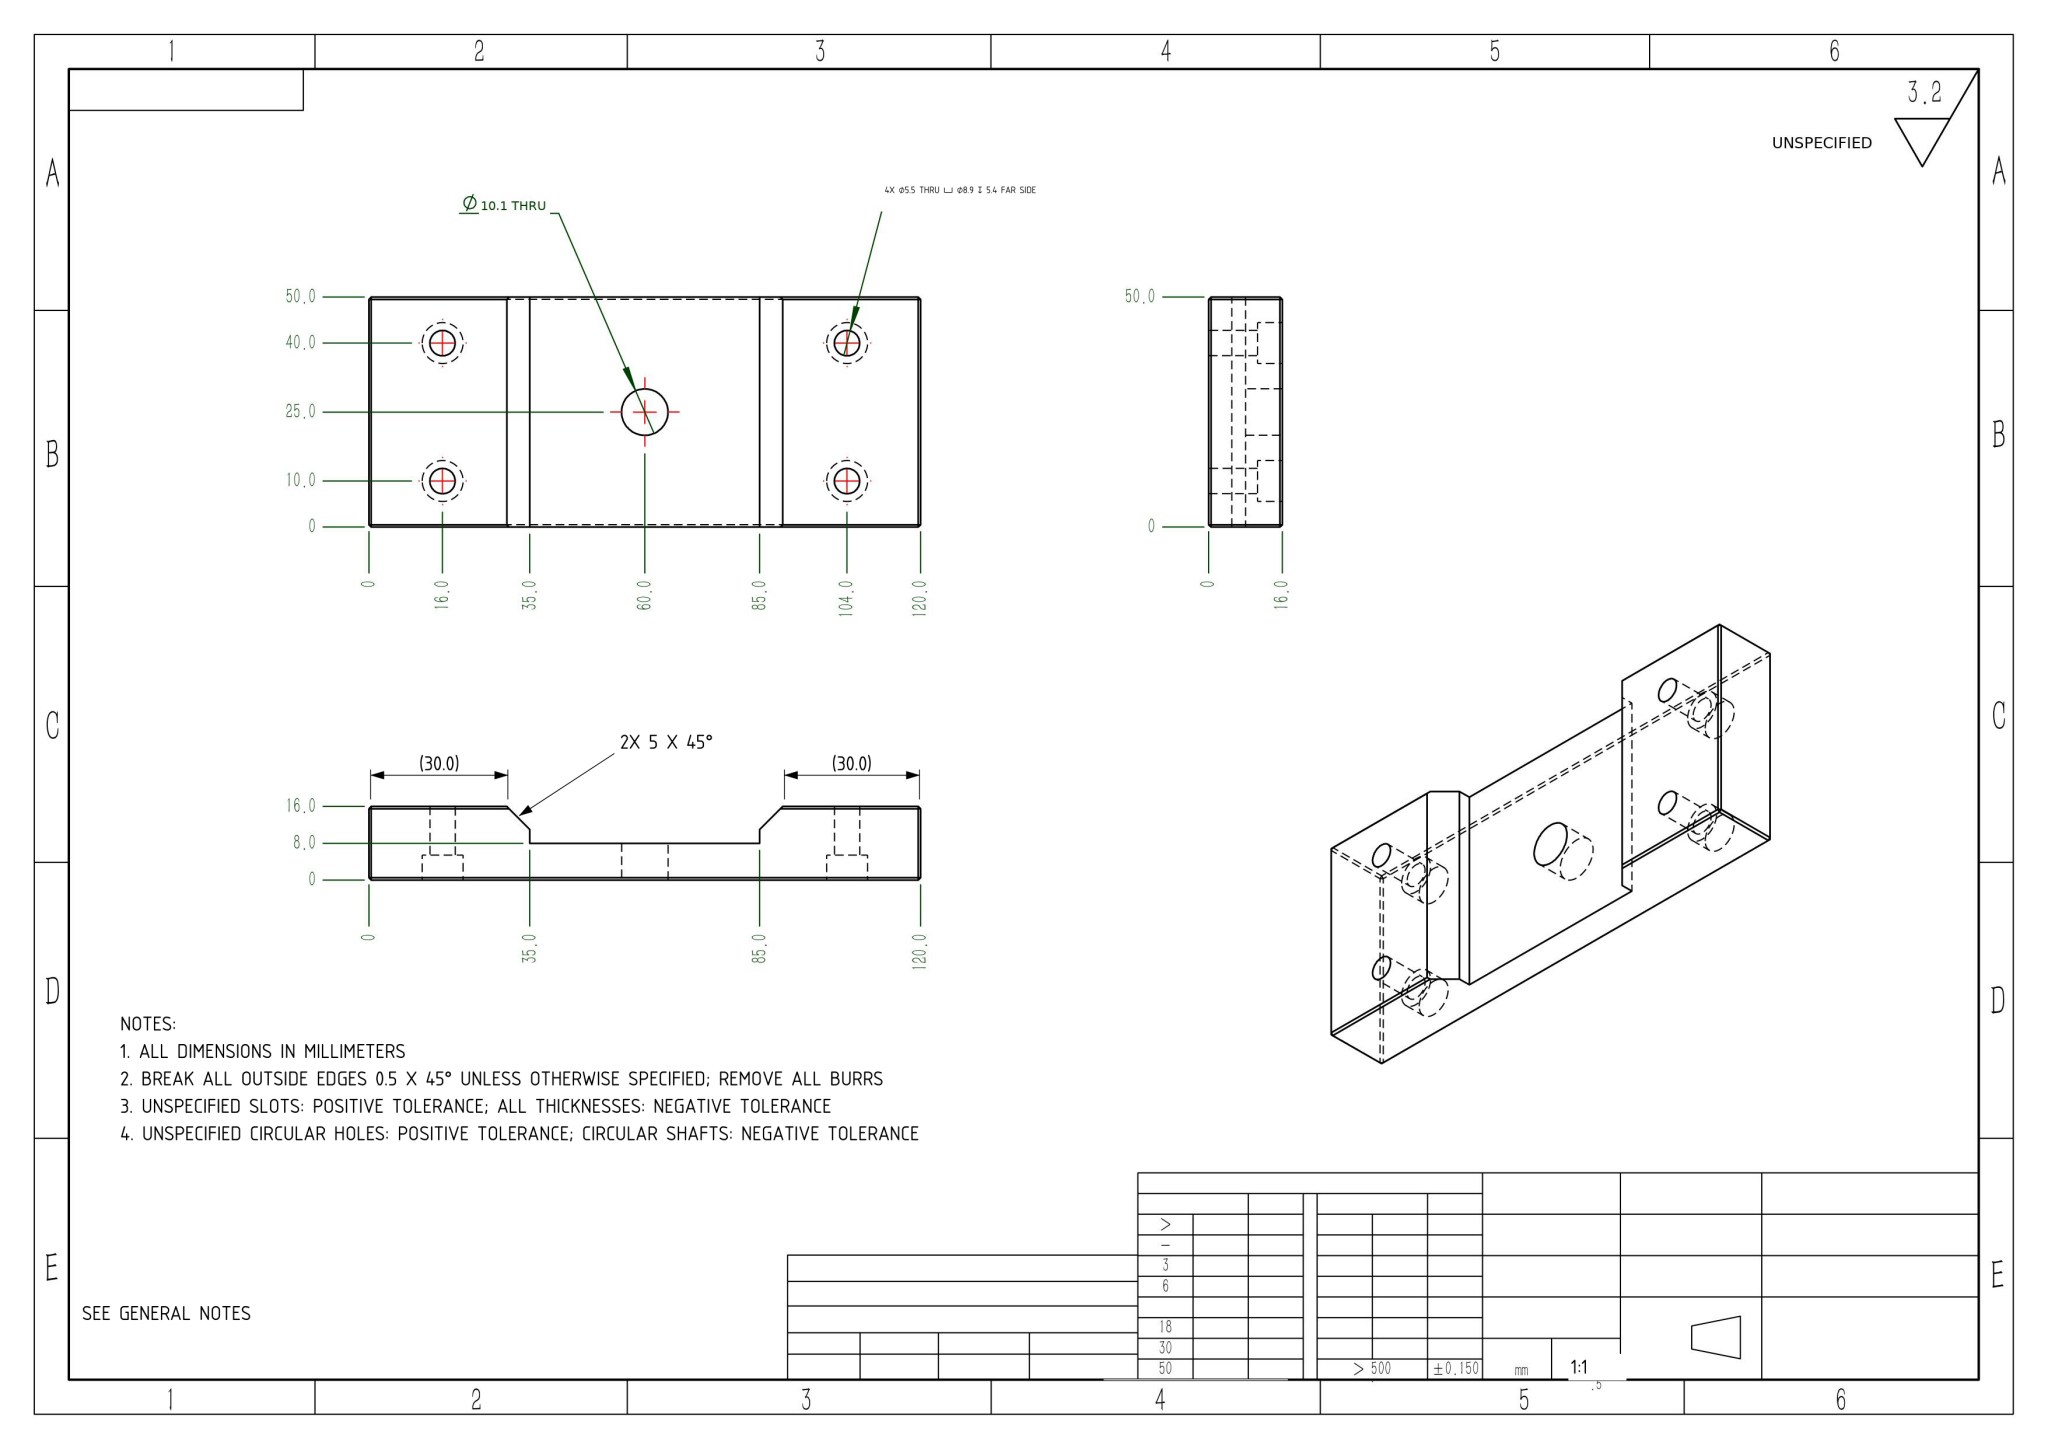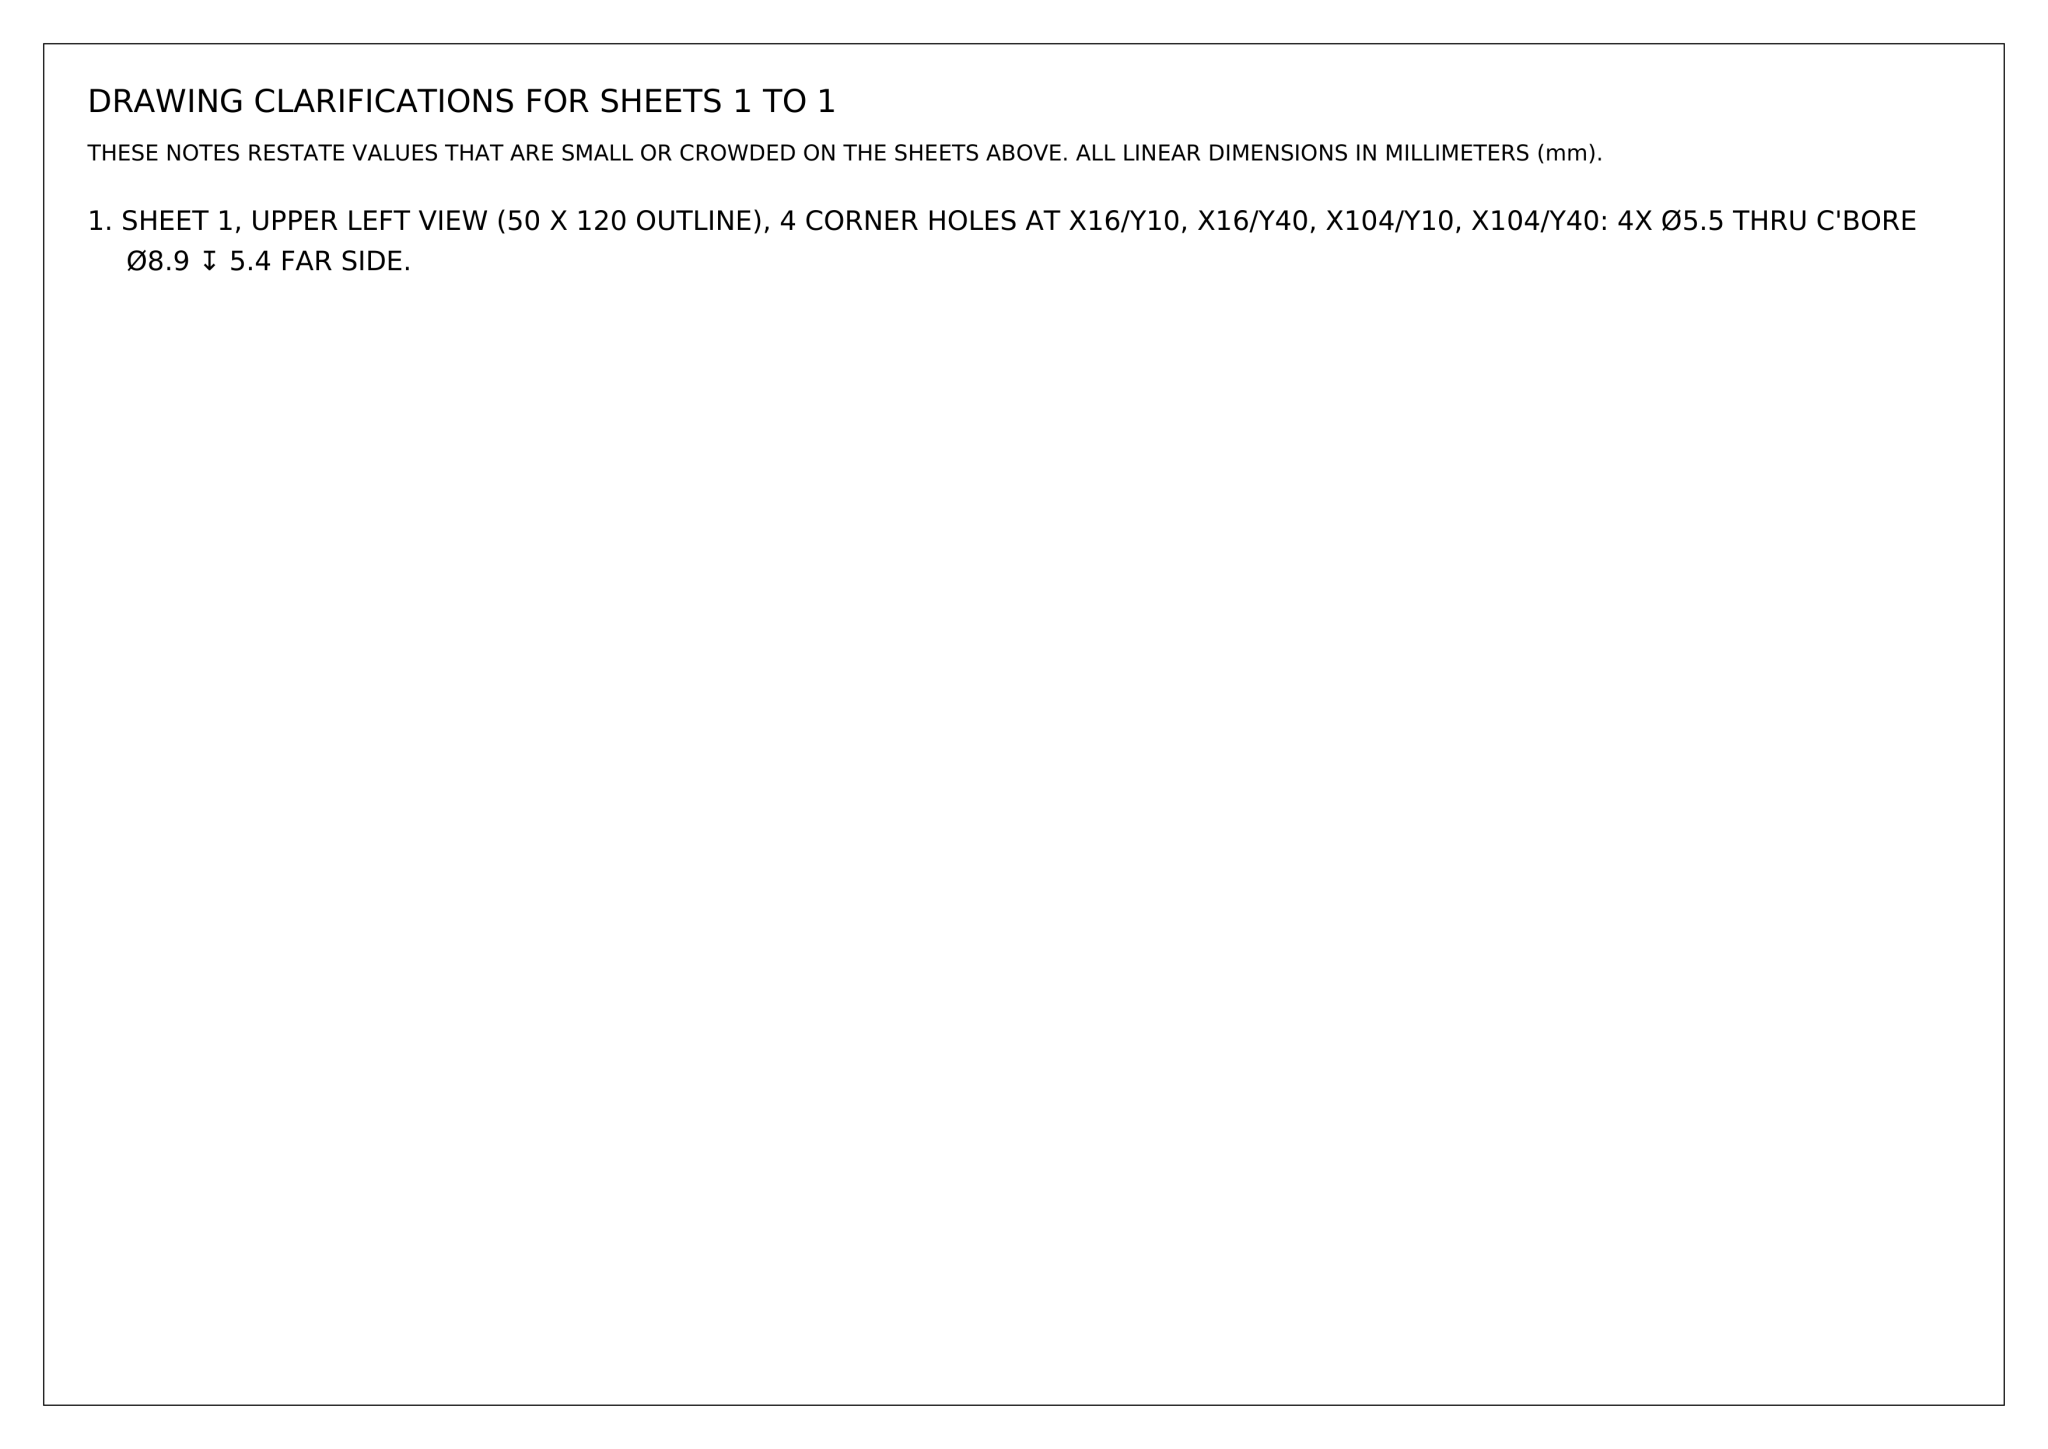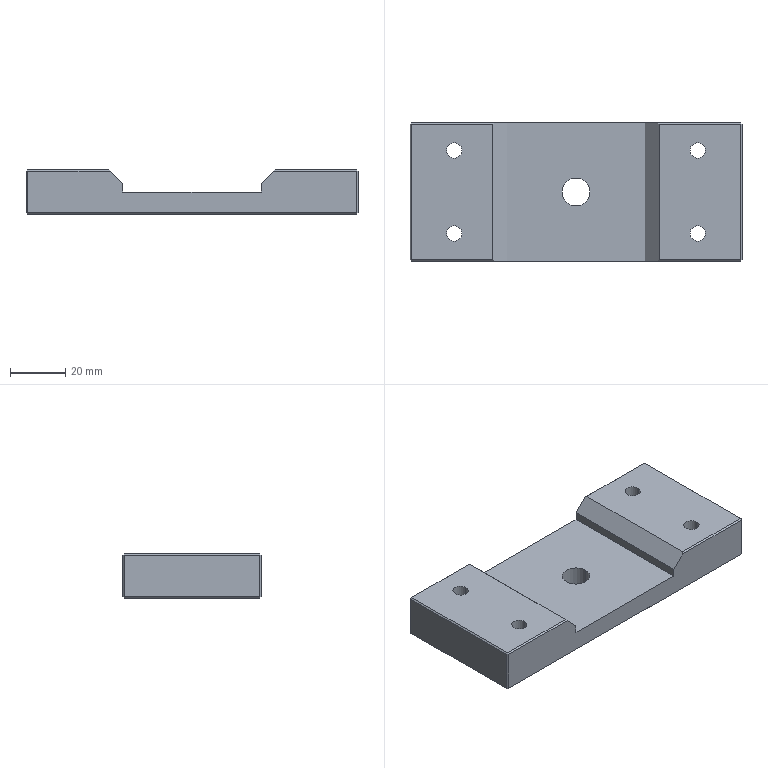Part | NX | mm | Stepped Multi-Bore Base Plate | 1 solid | 56 faces | box 120 x 50 x 16 mm | volume 71681 mm3 | plane 38 | cylinder 18 | commonest cylinder face diameters 8.9 x8 5.5 x8 10.1 x2